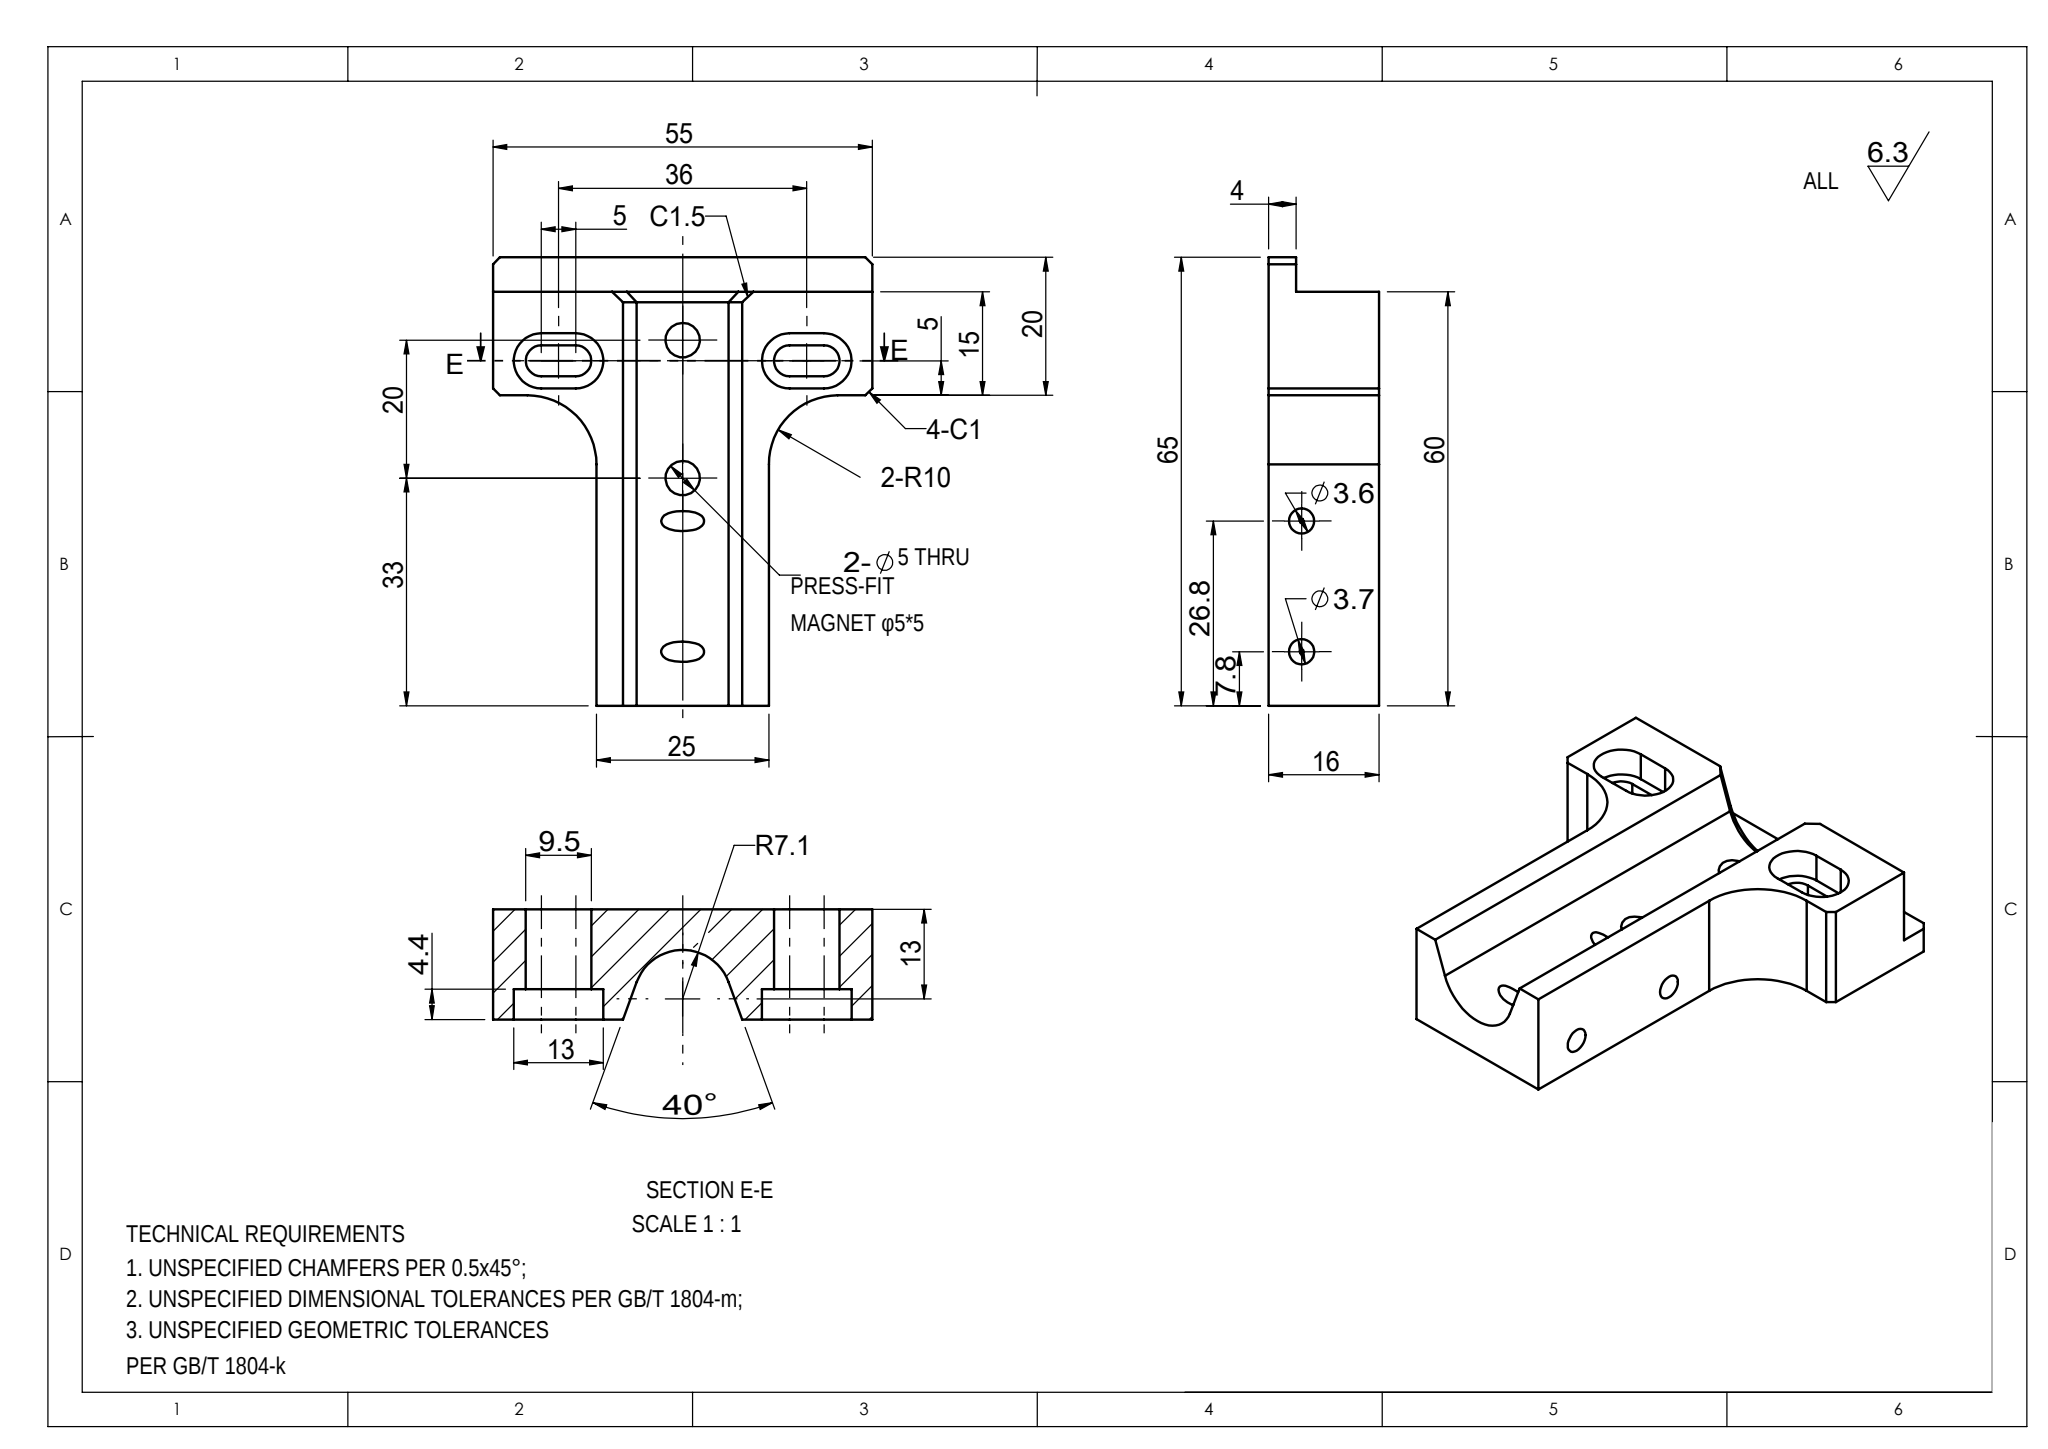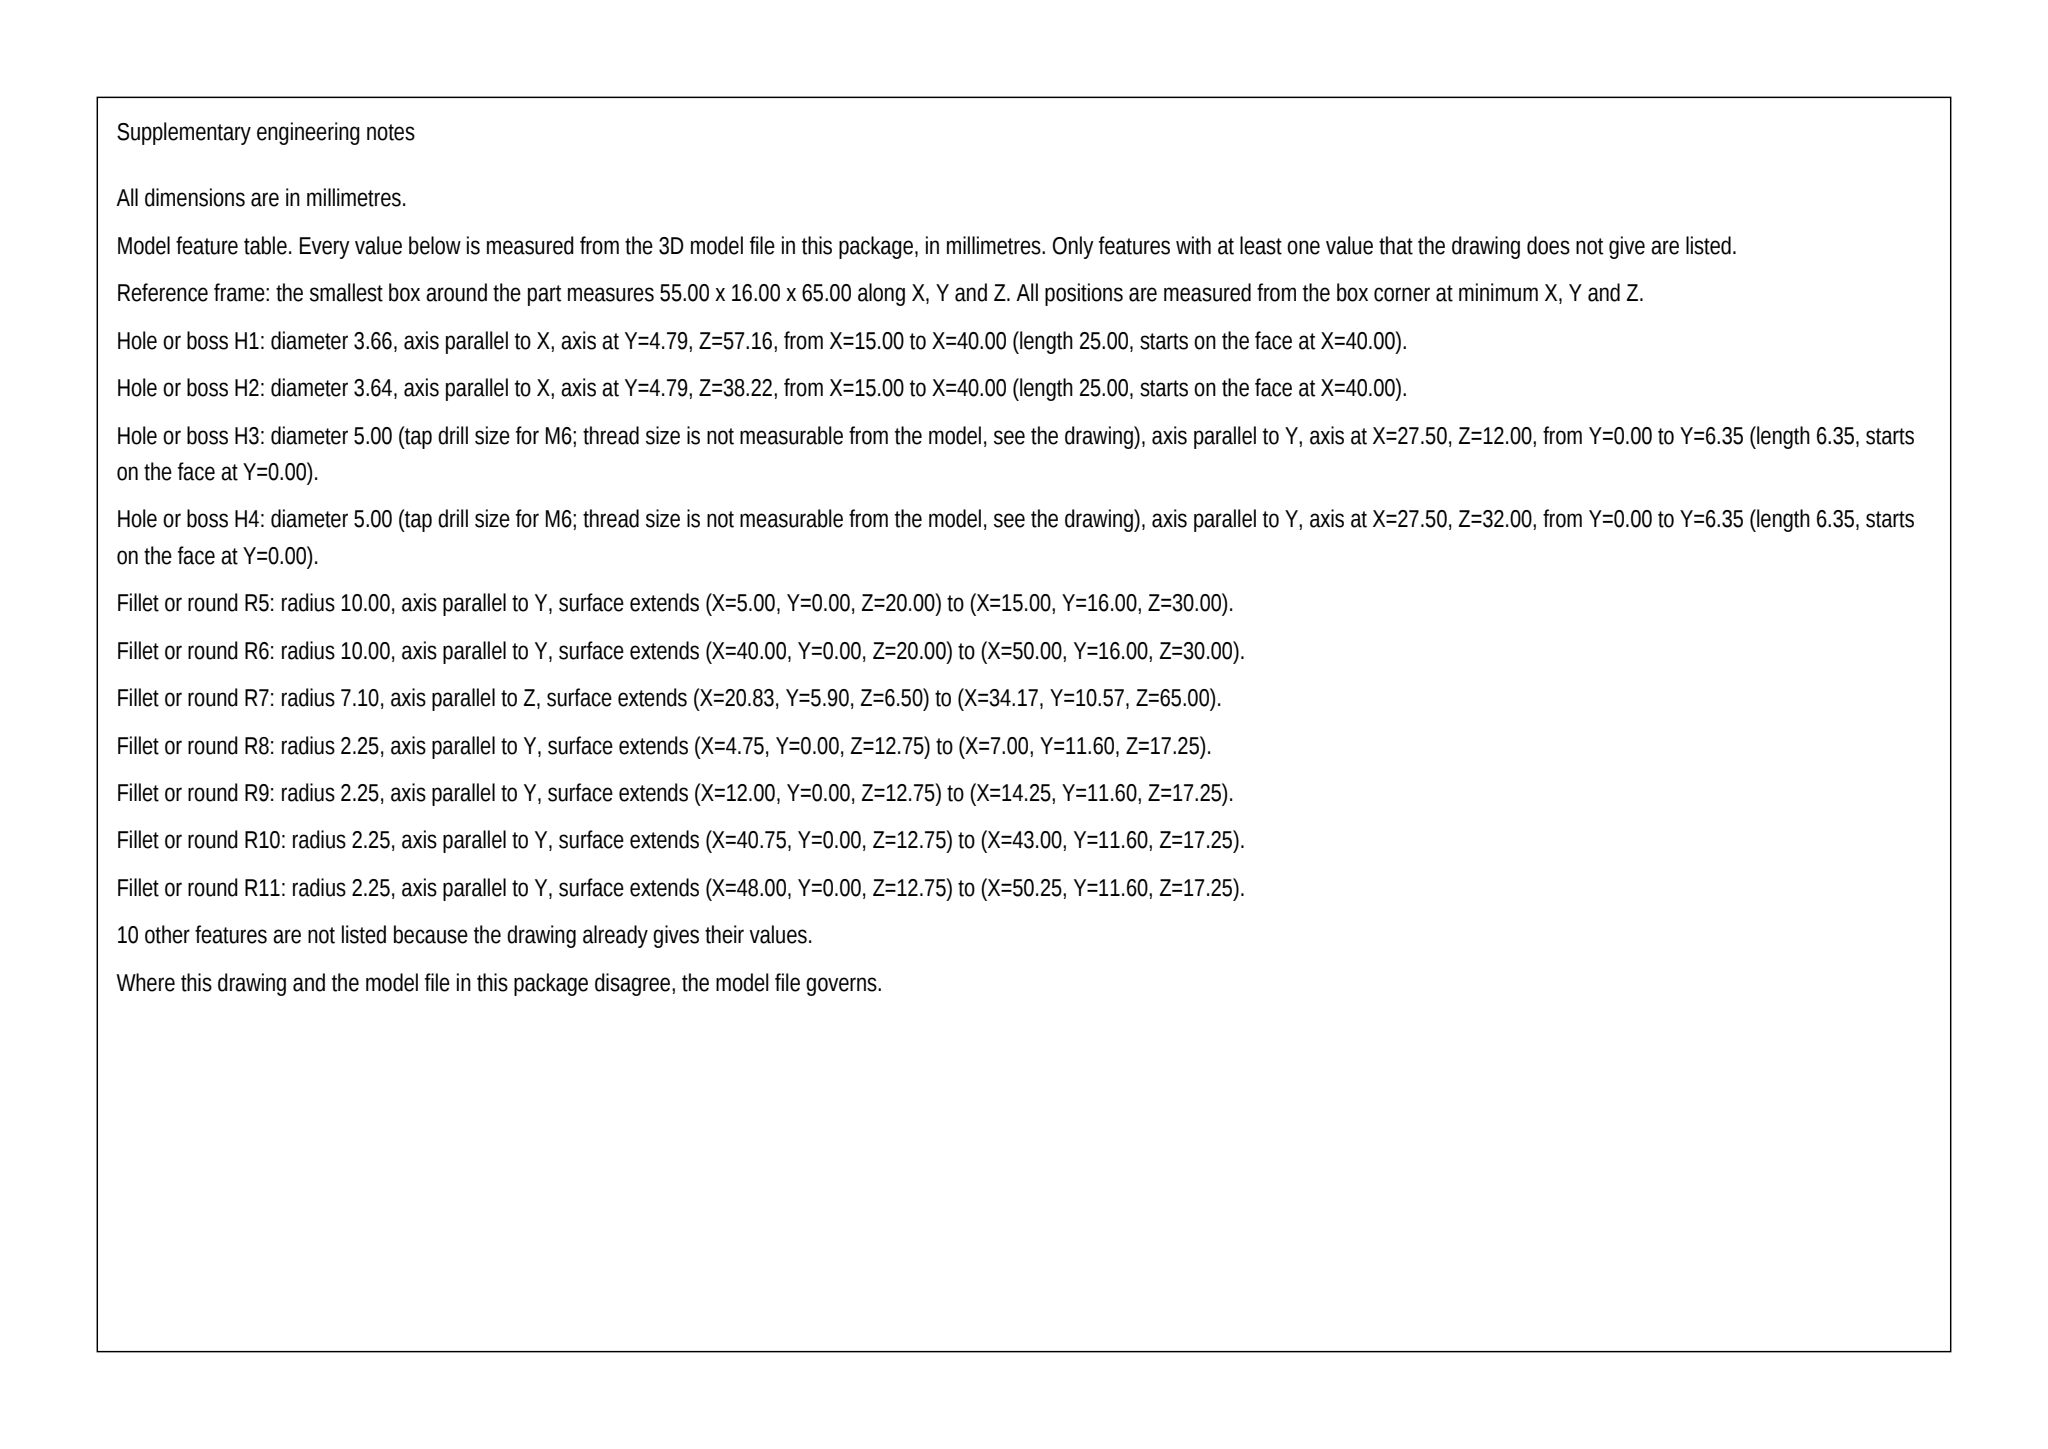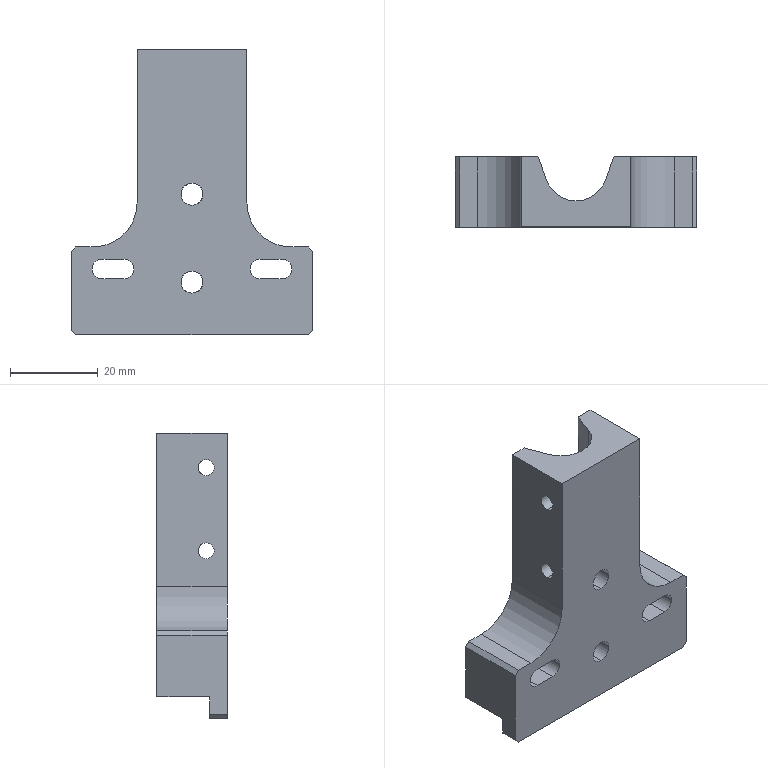Part | SolidWorks | mm | 1 solid | 51 faces | box 55 x 16 x 65 mm | volume 22785 mm3 | plane 31 | cylinder 19 | cone 1 | commonest cylinder face diameters 5 x4 4.5 x4 8 x4 3.663 x2 3.642 x2 20 x2 14.2 x1
build123d program:
from build123d import *

# Parameters (mm, degrees)
SKETCH1_W                                       = 25
SKETCH1_H                                       = 17
BOSS_EXTRUDE1_DEPTH                             = 65
CUT_EXTRUDE1_DEPTH                              = 70
SKETCH3_W                                       = 59.511
SKETCH3_H                                       = 18.848
CUT_EXTRUDE2_DEPTH                              = 80
SKETCH4_W                                       = 15
SKETCH4_H                                       = 20
BOSS_EXTRUDE2_DEPTH                             = 16
FILLET1_R                                       = 10
M4_HEX_SOCKET_HEAD_CAP_SCREW_CBORE1_D           = 4.5
M4_HEX_SOCKET_HEAD_CAP_SCREW_CBORE1_CBORE_D     = 8
M4_HEX_SOCKET_HEAD_CAP_SCREW_CBORE1_CBORE_DEPTH = 4.4
CHAMFER1_SIZE                                   = 1
CUT_EXTRUDE3_DEPTH                              = 4.4
CUT_EXTRUDE4_START                              = -30
CUT_EXTRUDE4_DEPTH                              = 30
SKETCH9_R                                       = 2.5
CUT_EXTRUDE5_DEPTH                              = 20
SKETCH10_W                                      = 73.82
SKETCH10_H                                      = 16.525
CUT_EXTRUDE6_DEPTH                              = 12
CHAMFER2_SIZE                                   = 1.5
SKETCH11_R                                      = 1.832
SKETCH11_R_2                                    = 1.821
CUT_EXTRUDE7_DEPTH                              = 80


with BuildPart() as part:
    # Sketch1 → Boss-Extrude1 (new body)
    with BuildSketch(Plane.XY):
        with Locations((-22.259, 32.627)):
            Rectangle(SKETCH1_W, SKETCH1_H)
    extrude(amount=BOSS_EXTRUDE1_DEPTH)

    # Sketch2 → Cut-Extrude1 (cut)
    with BuildSketch(Plane.XY.offset(65)):
        with BuildLine():
            Line((-31.27, 41.127), (-28.93, 34.699))
            ThreePointArc((-28.93, 34.699), (-22.259, 30.027), (-15.587, 34.699))
            Line((-15.587, 34.699), (-13.247, 41.127))
            Line((-13.247, 41.127), (-31.27, 41.127))
        make_face()
    extrude(amount=-CUT_EXTRUDE1_DEPTH, mode=Mode.SUBTRACT)

    # Sketch3 → Cut-Extrude2 (cut)
    with BuildSketch(Plane.XY.offset(65)):
        with Locations((-21.15, 49.551)):
            Rectangle(SKETCH3_W, SKETCH3_H)
    extrude(amount=-CUT_EXTRUDE2_DEPTH, mode=Mode.SUBTRACT)

    # Sketch4 → Boss-Extrude2 (add)
    with BuildSketch(Plane(origin=(0, 24.127, 0), x_dir=(1, 0, 0), z_dir=(0, 1, 0))):
        with Locations((-42.259, -10)):
            Rectangle(SKETCH4_W, SKETCH4_H)
        with Locations((-2.259, -10)):
            Rectangle(SKETCH4_W, SKETCH4_H)
    extrude(amount=BOSS_EXTRUDE2_DEPTH)

    # Fillet1
    fillet1_edges = [part.edges().sort_by_distance(p)[0] for p in [
        (-9.759, 32.127, 20),
        (-34.759, 32.127, 20),
    ]]
    fillet(fillet1_edges, radius=FILLET1_R)

    # M4 Hex Socket Head Cap Screw CBORE1 (through all)
    with Locations(Plane(origin=(0, 40.127, 0), x_dir=(1, 0, 0), z_dir=(0, 1, 0))):
        with Locations((-37.759, -15), (-6.759, -15)):
            CounterBoreHole(M4_HEX_SOCKET_HEAD_CAP_SCREW_CBORE1_D / 2, M4_HEX_SOCKET_HEAD_CAP_SCREW_CBORE1_CBORE_D / 2, M4_HEX_SOCKET_HEAD_CAP_SCREW_CBORE1_CBORE_DEPTH)

    # Chamfer1
    chamfer1_edges = [part.edges().sort_by_distance(p)[0] for p in [
        (5.241, 32.127, 20),
        (-49.759, 32.127, 20),
        (5.241, 32.127, 0),
        (-49.759, 32.127, 0),
    ]]
    chamfer(chamfer1_edges, length=CHAMFER1_SIZE)

    # Sketch7 → Cut-Extrude3 (cut)
    with BuildSketch(Plane(origin=(0, 40.127, 0), x_dir=(1, 0, 0), z_dir=(0, 1, 0))):
        with BuildLine():
            Line((-6.759, -11), (-1.759, -11))
            ThreePointArc((-1.759, -11), (2.241, -15), (-1.759, -19))
            Line((-1.759, -19), (-6.759, -19))
            ThreePointArc((-6.759, -19), (-10.759, -15), (-6.759, -11))
        make_face()
        with BuildLine():
            Line((-37.759, -11), (-42.759, -11))
            ThreePointArc((-42.759, -11), (-46.759, -15), (-42.759, -19))
            Line((-42.759, -19), (-37.759, -19))
            ThreePointArc((-37.759, -19), (-33.759, -15), (-37.759, -11))
        make_face()
    extrude(amount=-CUT_EXTRUDE3_DEPTH, mode=Mode.SUBTRACT)

    # Sketch8 → Cut-Extrude4 (cut)
    with BuildSketch(Plane(origin=(0, 35.727, 0), x_dir=(1, 0, 0), z_dir=(0, 1, 0)).offset(CUT_EXTRUDE4_START)):
        with BuildLine():
            Line((-6.759, -12.75), (-1.759, -12.75))
            ThreePointArc((-1.759, -12.75), (0.4914, -15), (-1.759, -17.25))
            Line((-1.759, -17.25), (-6.759, -17.25))
            ThreePointArc((-6.759, -17.25), (-9.009, -15), (-6.759, -12.75))
        make_face()
        with BuildLine():
            Line((-37.759, -17.25), (-42.759, -17.25))
            ThreePointArc((-42.759, -17.25), (-45.009, -15), (-42.759, -12.75))
            Line((-42.759, -12.75), (-37.759, -12.75))
            ThreePointArc((-37.759, -12.75), (-35.509, -15), (-37.759, -17.25))
        make_face()
    extrude(amount=CUT_EXTRUDE4_DEPTH, mode=Mode.SUBTRACT)

    # Sketch9 → Cut-Extrude5 (cut)
    with BuildSketch(Plane.XZ.offset(-24.127)):
        with Locations(Location((-22.259, 12, 0), (0, 0, 270))):
            Circle(SKETCH9_R)
        with Locations(Location((-22.259, 32, 0), (0, 0, 270))):
            Circle(SKETCH9_R)
    extrude(amount=-CUT_EXTRUDE5_DEPTH, mode=Mode.SUBTRACT)

    # Sketch10 → Cut-Extrude6 (cut)
    with BuildSketch(Plane(origin=(0, 40.127, 0), x_dir=(1, 0, 0), z_dir=(0, 1, 0))):
        with Locations((-23.931, 3.263)):
            Rectangle(SKETCH10_W, SKETCH10_H)
    extrude(amount=-CUT_EXTRUDE6_DEPTH, mode=Mode.SUBTRACT)

    # Chamfer2
    chamfer2_edges = [part.edges().sort_by_distance(p)[0] for p in [
        (-22.259, 30.027, 5),
        (-29.918, 37.413, 5),
        (-14.599, 37.413, 5),
    ]]
    chamfer(chamfer2_edges, length=CHAMFER2_SIZE)

    # Sketch11 → Cut-Extrude7 (cut)
    with BuildSketch(Plane(origin=(-9.759, 0, 0), x_dir=(0, 0, -1), z_dir=(1, 0, 0))):
        with Locations((-57.16, 28.917)):
            Circle(SKETCH11_R)
        with Locations((-38.217, 28.917)):
            Circle(SKETCH11_R_2)
    extrude(amount=-CUT_EXTRUDE7_DEPTH, mode=Mode.SUBTRACT)


solid = part.part